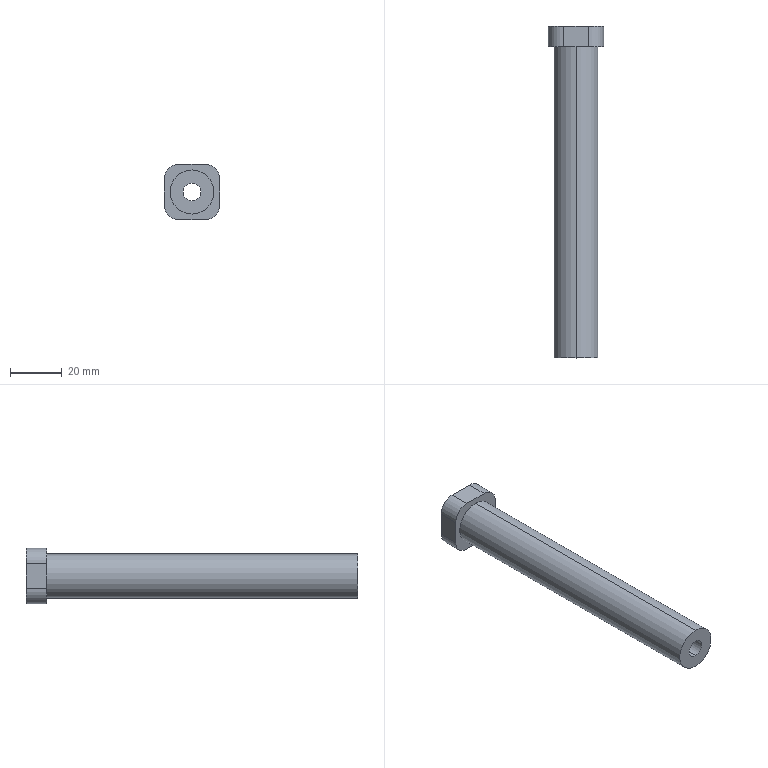CAM job | Mastercam | mm | 3 operations | part box 21.5 x 128 x 21.5
1. 2D High Speed (2D Dynamic Mill) | 10 - 10 平铣刀
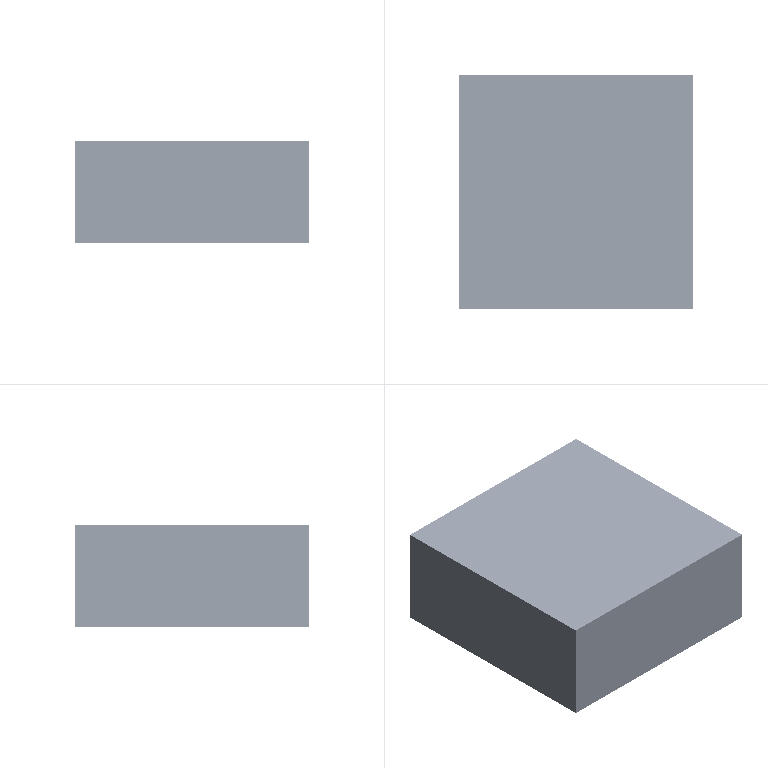2. Contour (2D) | 10 - 10 平铣刀
3. Contour (2D chamfer) | 7 - 4 倒角刀